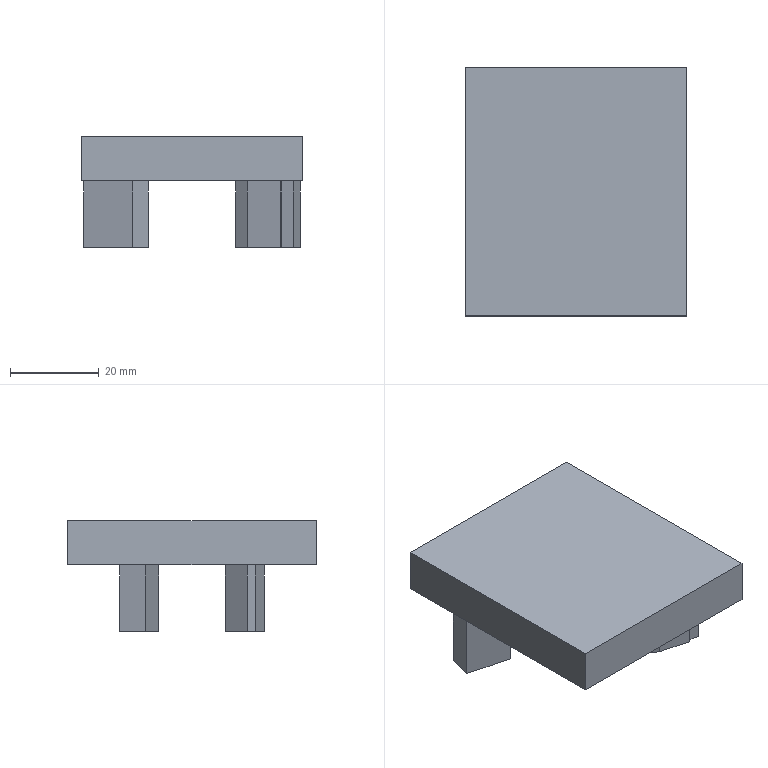Component | SolidWorks | 2023-12-12-30-1 | 1 solid | 22 faces | box 50 x 56 x 25 mm | volume 30440 mm3 | plane 22 | material S45C
build123d program:
from build123d import *

# Parameters (mm, degrees)
SKETCH1_W           = 50
SKETCH1_H           = 56
BOSS_EXTRUDE1_DEPTH = 25
SKETCH2_W           = 50
SKETCH2_H           = 56
CUT_EXTRUDE1_DEPTH  = 15


with BuildPart() as part:
    # Sketch1 → Boss-Extrude1 (new body)
    with BuildSketch(Plane.XY):
        with Locations((25, 28)):
            Rectangle(SKETCH1_W, SKETCH1_H)
    extrude(amount=BOSS_EXTRUDE1_DEPTH)

    # Sketch2 → Cut-Extrude1 (cut)
    with BuildSketch(Plane(origin=(0, 0, 0), x_dir=(-1, 0, 0), z_dir=(0, 0, -1))):
        with Locations((-25, 28)):
            Rectangle(SKETCH2_W, SKETCH2_H)
        Polygon((-44.917, 11.713), (-37.417, 13.723), (-34.917, 15.473), (-38.4, 20.447), (-49.4, 17.5), (-47.847, 11.704), (-45.111, 12.438), align=None, mode=Mode.SUBTRACT)
        Polygon((-4.889, 43.562), (-5.083, 44.287), (-12.583, 42.277), (-15.083, 40.527), (-11.6, 35.553), (-0.6, 38.5), (-2.153, 44.296), align=None, mode=Mode.SUBTRACT)
    extrude(amount=-CUT_EXTRUDE1_DEPTH, mode=Mode.SUBTRACT)


solid = part.part

# Placed as in the assembly
solid = solid.moved(Location((-93.778, -30.867, 92.891), (0, 0, 0)))
STEP:
#1=COLOUR_RGB('',0.7922,0.8196,0.9333);
#2=FILL_AREA_STYLE_COLOUR('',#1);
#3=FILL_AREA_STYLE('',(#2));
#4=SURFACE_STYLE_FILL_AREA(#3);
#5=SURFACE_SIDE_STYLE('',(#4));
#6=SURFACE_STYLE_USAGE(.BOTH.,#5);
#7=PRESENTATION_STYLE_ASSIGNMENT((#6));
#8=CARTESIAN_POINT('',(-3.692,0.9895,4.641));
#9=VERTEX_POINT('',#8);
#10=CARTESIAN_POINT('',(-3.692,0.9895,4.248));
#11=VERTEX_POINT('',#10);
#12=CARTESIAN_POINT('',(-3.692,0.9895,4.641));
#13=DIRECTION('',(0.,0.,-1.));
#14=VECTOR('',#13,39.37);
#15=LINE('',#12,#14);
#16=EDGE_CURVE('',#9,#11,#15,.T.);
#17=ORIENTED_EDGE('',*,*,#16,.T.);
#18=CARTESIAN_POINT('',(-3.692,-1.215,4.248));
#19=VERTEX_POINT('',#18);
#20=CARTESIAN_POINT('',(-3.692,-1.215,4.248));
#21=DIRECTION('',(0.,1.,0.));
#22=VECTOR('',#21,39.37);
#23=LINE('',#20,#22);
#24=EDGE_CURVE('',#19,#11,#23,.T.);
#25=ORIENTED_EDGE('',*,*,#24,.F.);
#26=CARTESIAN_POINT('',(-3.692,-1.215,4.641));
#27=VERTEX_POINT('',#26);
#28=CARTESIAN_POINT('',(-3.692,-1.215,4.641));
#29=DIRECTION('',(0.,0.,-1.));
#30=VECTOR('',#29,39.37);
#31=LINE('',#28,#30);
#32=EDGE_CURVE('',#27,#19,#31,.T.);
#33=ORIENTED_EDGE('',*,*,#32,.F.);
#34=CARTESIAN_POINT('',(-3.692,-1.215,4.641));
#35=DIRECTION('',(0.,-1.,0.));
#36=VECTOR('',#35,39.37);
#37=LINE('',#34,#36);
#38=EDGE_CURVE('',#9,#27,#37,.T.);
#39=ORIENTED_EDGE('',*,*,#38,.F.);
#40=EDGE_LOOP('',(#17,#25,#33,#39));
#41=FACE_OUTER_BOUND('',#40,.T.);
#42=CARTESIAN_POINT('',(-3.692,-1.215,4.641));
#43=DIRECTION('',(1.,0.,0.));
#44=DIRECTION('',(0.,0.,-1.));
#45=AXIS2_PLACEMENT_3D('',#42,#43,#44);
#46=PLANE('',#45);
#47=ADVANCED_FACE('',(#41),#46,.F.);
#48=ORIENTED_EDGE('',*,*,#32,.T.);
#49=CARTESIAN_POINT('',(-1.724,-1.215,4.248));
#50=VERTEX_POINT('',#49);
#51=CARTESIAN_POINT('',(-1.724,-1.215,4.248));
#52=DIRECTION('',(-1.,0.,0.));
#53=VECTOR('',#52,39.37);
#54=LINE('',#51,#53);
#55=EDGE_CURVE('',#50,#19,#54,.T.);
#56=ORIENTED_EDGE('',*,*,#55,.F.);
#57=CARTESIAN_POINT('',(-1.724,-1.215,4.641));
#58=VERTEX_POINT('',#57);
#59=CARTESIAN_POINT('',(-1.724,-1.215,4.641));
#60=DIRECTION('',(0.,0.,-1.));
#61=VECTOR('',#60,39.37);
#62=LINE('',#59,#61);
#63=EDGE_CURVE('',#58,#50,#62,.T.);
#64=ORIENTED_EDGE('',*,*,#63,.F.);
#65=CARTESIAN_POINT('',(-3.692,-1.215,4.641));
#66=DIRECTION('',(1.,0.,0.));
#67=VECTOR('',#66,39.37);
#68=LINE('',#65,#67);
#69=EDGE_CURVE('',#27,#58,#68,.T.);
#70=ORIENTED_EDGE('',*,*,#69,.F.);
#71=EDGE_LOOP('',(#48,#56,#64,#70));
#72=FACE_OUTER_BOUND('',#71,.T.);
#73=CARTESIAN_POINT('',(-3.692,-1.215,4.641));
#74=DIRECTION('',(0.,1.,0.));
#75=DIRECTION('',(0.,0.,1.));
#76=AXIS2_PLACEMENT_3D('',#73,#74,#75);
#77=PLANE('',#76);
#78=ADVANCED_FACE('',(#72),#77,.F.);
#79=ORIENTED_EDGE('',*,*,#63,.T.);
#80=CARTESIAN_POINT('',(-1.724,0.9895,4.248));
#81=VERTEX_POINT('',#80);
#82=CARTESIAN_POINT('',(-1.724,-1.215,4.248));
#83=DIRECTION('',(0.,-1.,0.));
#84=VECTOR('',#83,39.37);
#85=LINE('',#82,#84);
#86=EDGE_CURVE('',#81,#50,#85,.T.);
#87=ORIENTED_EDGE('',*,*,#86,.F.);
#88=CARTESIAN_POINT('',(-1.724,0.9895,4.641));
#89=VERTEX_POINT('',#88);
#90=CARTESIAN_POINT('',(-1.724,0.9895,4.641));
#91=DIRECTION('',(0.,0.,-1.));
#92=VECTOR('',#91,39.37);
#93=LINE('',#90,#92);
#94=EDGE_CURVE('',#89,#81,#93,.T.);
#95=ORIENTED_EDGE('',*,*,#94,.F.);
#96=CARTESIAN_POINT('',(-1.724,-1.215,4.641));
#97=DIRECTION('',(0.,1.,0.));
#98=VECTOR('',#97,39.37);
#99=LINE('',#96,#98);
#100=EDGE_CURVE('',#58,#89,#99,.T.);
#101=ORIENTED_EDGE('',*,*,#100,.F.);
#102=EDGE_LOOP('',(#79,#87,#95,#101));
#103=FACE_OUTER_BOUND('',#102,.T.);
#104=CARTESIAN_POINT('',(-1.724,-1.215,4.641));
#105=DIRECTION('',(-1.,0.,0.));
#106=DIRECTION('',(0.,0.,1.));
#107=AXIS2_PLACEMENT_3D('',#104,#105,#106);
#108=PLANE('',#107);
#109=ADVANCED_FACE('',(#103),#108,.F.);
#110=ORIENTED_EDGE('',*,*,#94,.T.);
#111=CARTESIAN_POINT('',(-1.724,0.9895,4.248));
#112=DIRECTION('',(1.,0.,0.));
#113=VECTOR('',#112,39.37);
#114=LINE('',#111,#113);
#115=EDGE_CURVE('',#11,#81,#114,.T.);
#116=ORIENTED_EDGE('',*,*,#115,.F.);
#117=ORIENTED_EDGE('',*,*,#16,.F.);
#118=CARTESIAN_POINT('',(-3.692,0.9895,4.641));
#119=DIRECTION('',(-1.,0.,0.));
#120=VECTOR('',#119,39.37);
#121=LINE('',#118,#120);
#122=EDGE_CURVE('',#89,#9,#121,.T.);
#123=ORIENTED_EDGE('',*,*,#122,.F.);
#124=EDGE_LOOP('',(#110,#116,#117,#123));
#125=FACE_OUTER_BOUND('',#124,.T.);
#126=CARTESIAN_POINT('',(-3.692,0.9895,4.641));
#127=DIRECTION('',(0.,-1.,0.));
#128=DIRECTION('',(0.,0.,-1.));
#129=AXIS2_PLACEMENT_3D('',#126,#127,#128);
#130=PLANE('',#129);
#131=ADVANCED_FACE('',(#125),#130,.F.);
#132=ORIENTED_EDGE('',*,*,#38,.T.);
#133=ORIENTED_EDGE('',*,*,#69,.T.);
#134=ORIENTED_EDGE('',*,*,#100,.T.);
#135=ORIENTED_EDGE('',*,*,#122,.T.);
#136=EDGE_LOOP('',(#132,#133,#134,#135));
#137=FACE_OUTER_BOUND('',#136,.T.);
#138=CARTESIAN_POINT('',(-3.692,-1.215,4.641));
#139=DIRECTION('',(0.,0.,-1.));
#140=DIRECTION('',(-1.,0.,0.));
#141=AXIS2_PLACEMENT_3D('',#138,#139,#140);
#142=PLANE('',#141);
#143=ADVANCED_FACE('',(#137),#142,.F.);
#144=CARTESIAN_POINT('',(-3.492,0.5284,4.248));
#145=VERTEX_POINT('',#144);
#146=CARTESIAN_POINT('',(-3.197,0.4492,4.248));
#147=VERTEX_POINT('',#146);
#148=CARTESIAN_POINT('',(-3.492,0.5284,4.248));
#149=DIRECTION('',(0.9659,-0.2588,0.));
#150=VECTOR('',#149,39.37);
#151=LINE('',#148,#150);
#152=EDGE_CURVE('',#145,#147,#151,.T.);
#153=ORIENTED_EDGE('',*,*,#152,.F.);
#154=CARTESIAN_POINT('',(-3.5,0.4998,4.248));
#155=VERTEX_POINT('',#154);
#156=CARTESIAN_POINT('',(-3.5,0.4998,4.248));
#157=DIRECTION('',(0.2588,0.9659,0.));
#158=VECTOR('',#157,39.37);
#159=LINE('',#156,#158);
#160=EDGE_CURVE('',#155,#145,#159,.T.);
#161=ORIENTED_EDGE('',*,*,#160,.F.);
#162=CARTESIAN_POINT('',(-3.607,0.5287,4.248));
#163=VERTEX_POINT('',#162);
#164=CARTESIAN_POINT('',(-3.607,0.5287,4.248));
#165=DIRECTION('',(0.9659,-0.2588,0.));
#166=VECTOR('',#165,39.37);
#167=LINE('',#164,#166);
#168=EDGE_CURVE('',#163,#155,#167,.T.);
#169=ORIENTED_EDGE('',*,*,#168,.F.);
#170=CARTESIAN_POINT('',(-3.668,0.3005,4.248));
#171=VERTEX_POINT('',#170);
#172=CARTESIAN_POINT('',(-3.668,0.3005,4.248));
#173=DIRECTION('',(0.2588,0.9659,0.));
#174=VECTOR('',#173,39.37);
#175=LINE('',#172,#174);
#176=EDGE_CURVE('',#171,#163,#175,.T.);
#177=ORIENTED_EDGE('',*,*,#176,.F.);
#178=CARTESIAN_POINT('',(-3.235,0.1845,4.248));
#179=VERTEX_POINT('',#178);
#180=CARTESIAN_POINT('',(-3.235,0.1845,4.248));
#181=DIRECTION('',(-0.9659,0.2588,0.));
#182=VECTOR('',#181,39.37);
#183=LINE('',#180,#182);
#184=EDGE_CURVE('',#179,#171,#183,.T.);
#185=ORIENTED_EDGE('',*,*,#184,.F.);
#186=CARTESIAN_POINT('',(-3.098,0.3803,4.248));
#187=VERTEX_POINT('',#186);
#188=CARTESIAN_POINT('',(-3.098,0.3803,4.248));
#189=DIRECTION('',(-0.5736,-0.8192,0.));
#190=VECTOR('',#189,39.37);
#191=LINE('',#188,#190);
#192=EDGE_CURVE('',#187,#179,#191,.T.);
#193=ORIENTED_EDGE('',*,*,#192,.F.);
#194=CARTESIAN_POINT('',(-3.197,0.4492,4.248));
#195=DIRECTION('',(0.8192,-0.5736,0.));
#196=VECTOR('',#195,39.37);
#197=LINE('',#194,#196);
#198=EDGE_CURVE('',#147,#187,#197,.T.);
#199=ORIENTED_EDGE('',*,*,#198,.F.);
#200=EDGE_LOOP('',(#153,#161,#169,#177,#185,#193,#199));
#201=FACE_BOUND('',#200,.T.);
#202=CARTESIAN_POINT('',(-1.916,-0.7256,4.248));
#203=VERTEX_POINT('',#202);
#204=CARTESIAN_POINT('',(-1.924,-0.7541,4.248));
#205=VERTEX_POINT('',#204);
#206=CARTESIAN_POINT('',(-1.916,-0.7256,4.248));
#207=DIRECTION('',(-0.2588,-0.9659,0.));
#208=VECTOR('',#207,39.37);
#209=LINE('',#206,#208);
#210=EDGE_CURVE('',#203,#205,#209,.T.);
#211=ORIENTED_EDGE('',*,*,#210,.F.);
#212=CARTESIAN_POINT('',(-1.808,-0.7544,4.248));
#213=VERTEX_POINT('',#212);
#214=CARTESIAN_POINT('',(-1.808,-0.7544,4.248));
#215=DIRECTION('',(-0.9659,0.2588,0.));
#216=VECTOR('',#215,39.37);
#217=LINE('',#214,#216);
#218=EDGE_CURVE('',#213,#203,#217,.T.);
#219=ORIENTED_EDGE('',*,*,#218,.F.);
#220=CARTESIAN_POINT('',(-1.747,-0.5262,4.248));
#221=VERTEX_POINT('',#220);
#222=CARTESIAN_POINT('',(-1.747,-0.5262,4.248));
#223=DIRECTION('',(-0.2588,-0.9659,0.));
#224=VECTOR('',#223,39.37);
#225=LINE('',#222,#224);
#226=EDGE_CURVE('',#221,#213,#225,.T.);
#227=ORIENTED_EDGE('',*,*,#226,.F.);
#228=CARTESIAN_POINT('',(-2.18,-0.4102,4.248));
#229=VERTEX_POINT('',#228);
#230=CARTESIAN_POINT('',(-2.18,-0.4102,4.248));
#231=DIRECTION('',(0.9659,-0.2588,0.));
#232=VECTOR('',#231,39.37);
#233=LINE('',#230,#232);
#234=EDGE_CURVE('',#229,#221,#233,.T.);
#235=ORIENTED_EDGE('',*,*,#234,.F.);
#236=CARTESIAN_POINT('',(-2.317,-0.606,4.248));
#237=VERTEX_POINT('',#236);
#238=CARTESIAN_POINT('',(-2.317,-0.606,4.248));
#239=DIRECTION('',(0.5736,0.8192,0.));
#240=VECTOR('',#239,39.37);
#241=LINE('',#238,#240);
#242=EDGE_CURVE('',#237,#229,#241,.T.);
#243=ORIENTED_EDGE('',*,*,#242,.F.);
#244=CARTESIAN_POINT('',(-2.219,-0.675,4.248));
#245=VERTEX_POINT('',#244);
#246=CARTESIAN_POINT('',(-2.219,-0.675,4.248));
#247=DIRECTION('',(-0.8192,0.5736,0.));
#248=VECTOR('',#247,39.37);
#249=LINE('',#246,#248);
#250=EDGE_CURVE('',#245,#237,#249,.T.);
#251=ORIENTED_EDGE('',*,*,#250,.F.);
#252=CARTESIAN_POINT('',(-1.924,-0.7541,4.248));
#253=DIRECTION('',(-0.9659,0.2588,0.));
#254=VECTOR('',#253,39.37);
#255=LINE('',#252,#254);
#256=EDGE_CURVE('',#205,#245,#255,.T.);
#257=ORIENTED_EDGE('',*,*,#256,.F.);
#258=EDGE_LOOP('',(#211,#219,#227,#235,#243,#251,#257));
#259=FACE_BOUND('',#258,.T.);
#260=ORIENTED_EDGE('',*,*,#86,.T.);
#261=ORIENTED_EDGE('',*,*,#55,.T.);
#262=ORIENTED_EDGE('',*,*,#24,.T.);
#263=ORIENTED_EDGE('',*,*,#115,.T.);
#264=EDGE_LOOP('',(#260,#261,#262,#263));
#265=FACE_OUTER_BOUND('',#264,.T.);
#266=CARTESIAN_POINT('',(-3.692,-1.215,4.248));
#267=DIRECTION('',(0.,0.,1.));
#268=DIRECTION('',(1.,0.,0.));
#269=AXIS2_PLACEMENT_3D('',#266,#267,#268);
#270=PLANE('',#269);
#271=ADVANCED_FACE('',(#201,#259,#265),#270,.F.);
#272=CARTESIAN_POINT('',(-1.916,-0.7256,3.657));
#273=VERTEX_POINT('',#272);
#274=CARTESIAN_POINT('',(-1.924,-0.7541,3.657));
#275=VERTEX_POINT('',#274);
#276=CARTESIAN_POINT('',(-1.916,-0.7256,3.657));
#277=DIRECTION('',(-0.2588,-0.9659,0.));
#278=VECTOR('',#277,39.37);
#279=LINE('',#276,#278);
#280=EDGE_CURVE('',#273,#275,#279,.T.);
#281=ORIENTED_EDGE('',*,*,#280,.F.);
#282=CARTESIAN_POINT('',(-1.916,-0.7256,4.248));
#283=DIRECTION('',(0.,0.,-1.));
#284=VECTOR('',#283,39.37);
#285=LINE('',#282,#284);
#286=EDGE_CURVE('',#203,#273,#285,.T.);
#287=ORIENTED_EDGE('',*,*,#286,.F.);
#288=ORIENTED_EDGE('',*,*,#210,.T.);
#289=CARTESIAN_POINT('',(-1.924,-0.7541,4.248));
#290=DIRECTION('',(0.,0.,-1.));
#291=VECTOR('',#290,39.37);
#292=LINE('',#289,#291);
#293=EDGE_CURVE('',#205,#275,#292,.T.);
#294=ORIENTED_EDGE('',*,*,#293,.T.);
#295=EDGE_LOOP('',(#281,#287,#288,#294));
#296=FACE_OUTER_BOUND('',#295,.T.);
#297=CARTESIAN_POINT('',(-1.916,-0.7256,4.248));
#298=DIRECTION('',(0.9659,-0.2588,0.));
#299=DIRECTION('',(0.2588,0.9659,0.));
#300=AXIS2_PLACEMENT_3D('',#297,#298,#299);
#301=PLANE('',#300);
#302=ADVANCED_FACE('',(#296),#301,.T.);
#303=CARTESIAN_POINT('',(-1.808,-0.7544,3.657));
#304=VERTEX_POINT('',#303);
#305=CARTESIAN_POINT('',(-1.808,-0.7544,3.657));
#306=DIRECTION('',(-0.9659,0.2588,0.));
#307=VECTOR('',#306,39.37);
#308=LINE('',#305,#307);
#309=EDGE_CURVE('',#304,#273,#308,.T.);
#310=ORIENTED_EDGE('',*,*,#309,.F.);
#311=CARTESIAN_POINT('',(-1.808,-0.7544,4.248));
#312=DIRECTION('',(0.,0.,-1.));
#313=VECTOR('',#312,39.37);
#314=LINE('',#311,#313);
#315=EDGE_CURVE('',#213,#304,#314,.T.);
#316=ORIENTED_EDGE('',*,*,#315,.F.);
#317=ORIENTED_EDGE('',*,*,#218,.T.);
#318=ORIENTED_EDGE('',*,*,#286,.T.);
#319=EDGE_LOOP('',(#310,#316,#317,#318));
#320=FACE_OUTER_BOUND('',#319,.T.);
#321=CARTESIAN_POINT('',(-1.808,-0.7544,4.248));
#322=DIRECTION('',(-0.2588,-0.9659,0.));
#323=DIRECTION('',(0.9659,-0.2588,0.));
#324=AXIS2_PLACEMENT_3D('',#321,#322,#323);
#325=PLANE('',#324);
#326=ADVANCED_FACE('',(#320),#325,.T.);
#327=CARTESIAN_POINT('',(-1.747,-0.5262,3.657));
#328=VERTEX_POINT('',#327);
#329=CARTESIAN_POINT('',(-1.747,-0.5262,3.657));
#330=DIRECTION('',(-0.2588,-0.9659,0.));
#331=VECTOR('',#330,39.37);
#332=LINE('',#329,#331);
#333=EDGE_CURVE('',#328,#304,#332,.T.);
#334=ORIENTED_EDGE('',*,*,#333,.F.);
#335=CARTESIAN_POINT('',(-1.747,-0.5262,4.248));
#336=DIRECTION('',(0.,0.,-1.));
#337=VECTOR('',#336,39.37);
#338=LINE('',#335,#337);
#339=EDGE_CURVE('',#221,#328,#338,.T.);
#340=ORIENTED_EDGE('',*,*,#339,.F.);
#341=ORIENTED_EDGE('',*,*,#226,.T.);
#342=ORIENTED_EDGE('',*,*,#315,.T.);
#343=EDGE_LOOP('',(#334,#340,#341,#342));
#344=FACE_OUTER_BOUND('',#343,.T.);
#345=CARTESIAN_POINT('',(-1.747,-0.5262,4.248));
#346=DIRECTION('',(0.9659,-0.2588,0.));
#347=DIRECTION('',(0.2588,0.9659,0.));
#348=AXIS2_PLACEMENT_3D('',#345,#346,#347);
#349=PLANE('',#348);
#350=ADVANCED_FACE('',(#344),#349,.T.);
#351=CARTESIAN_POINT('',(-2.18,-0.4102,3.657));
#352=VERTEX_POINT('',#351);
#353=CARTESIAN_POINT('',(-2.18,-0.4102,3.657));
#354=DIRECTION('',(0.9659,-0.2588,0.));
#355=VECTOR('',#354,39.37);
#356=LINE('',#353,#355);
#357=EDGE_CURVE('',#352,#328,#356,.T.);
#358=ORIENTED_EDGE('',*,*,#357,.F.);
#359=CARTESIAN_POINT('',(-2.18,-0.4102,4.248));
#360=DIRECTION('',(0.,0.,-1.));
#361=VECTOR('',#360,39.37);
#362=LINE('',#359,#361);
#363=EDGE_CURVE('',#229,#352,#362,.T.);
#364=ORIENTED_EDGE('',*,*,#363,.F.);
#365=ORIENTED_EDGE('',*,*,#234,.T.);
#366=ORIENTED_EDGE('',*,*,#339,.T.);
#367=EDGE_LOOP('',(#358,#364,#365,#366));
#368=FACE_OUTER_BOUND('',#367,.T.);
#369=CARTESIAN_POINT('',(-2.18,-0.4102,4.248));
#370=DIRECTION('',(0.2588,0.9659,0.));
#371=DIRECTION('',(-0.9659,0.2588,0.));
#372=AXIS2_PLACEMENT_3D('',#369,#370,#371);
#373=PLANE('',#372);
#374=ADVANCED_FACE('',(#368),#373,.T.);
#375=CARTESIAN_POINT('',(-2.317,-0.606,3.657));
#376=VERTEX_POINT('',#375);
#377=CARTESIAN_POINT('',(-2.317,-0.606,3.657));
#378=DIRECTION('',(0.5736,0.8192,0.));
#379=VECTOR('',#378,39.37);
#380=LINE('',#377,#379);
#381=EDGE_CURVE('',#376,#352,#380,.T.);
#382=ORIENTED_EDGE('',*,*,#381,.F.);
#383=CARTESIAN_POINT('',(-2.317,-0.606,4.248));
#384=DIRECTION('',(0.,0.,-1.));
#385=VECTOR('',#384,39.37);
#386=LINE('',#383,#385);
#387=EDGE_CURVE('',#237,#376,#386,.T.);
#388=ORIENTED_EDGE('',*,*,#387,.F.);
#389=ORIENTED_EDGE('',*,*,#242,.T.);
#390=ORIENTED_EDGE('',*,*,#363,.T.);
#391=EDGE_LOOP('',(#382,#388,#389,#390));
#392=FACE_OUTER_BOUND('',#391,.T.);
#393=CARTESIAN_POINT('',(-2.317,-0.606,4.248));
#394=DIRECTION('',(-0.8192,0.5736,0.));
#395=DIRECTION('',(-0.5736,-0.8192,0.));
#396=AXIS2_PLACEMENT_3D('',#393,#394,#395);
#397=PLANE('',#396);
#398=ADVANCED_FACE('',(#392),#397,.T.);
#399=CARTESIAN_POINT('',(-2.219,-0.675,3.657));
#400=VERTEX_POINT('',#399);
#401=CARTESIAN_POINT('',(-2.219,-0.675,3.657));
#402=DIRECTION('',(-0.8192,0.5736,0.));
#403=VECTOR('',#402,39.37);
#404=LINE('',#401,#403);
#405=EDGE_CURVE('',#400,#376,#404,.T.);
#406=ORIENTED_EDGE('',*,*,#405,.F.);
#407=CARTESIAN_POINT('',(-2.219,-0.675,4.248));
#408=DIRECTION('',(0.,0.,-1.));
#409=VECTOR('',#408,39.37);
#410=LINE('',#407,#409);
#411=EDGE_CURVE('',#245,#400,#410,.T.);
#412=ORIENTED_EDGE('',*,*,#411,.F.);
#413=ORIENTED_EDGE('',*,*,#250,.T.);
#414=ORIENTED_EDGE('',*,*,#387,.T.);
#415=EDGE_LOOP('',(#406,#412,#413,#414));
#416=FACE_OUTER_BOUND('',#415,.T.);
#417=CARTESIAN_POINT('',(-2.219,-0.675,4.248));
#418=DIRECTION('',(-0.5736,-0.8192,0.));
#419=DIRECTION('',(0.8192,-0.5736,0.));
#420=AXIS2_PLACEMENT_3D('',#417,#418,#419);
#421=PLANE('',#420);
#422=ADVANCED_FACE('',(#416),#421,.T.);
#423=CARTESIAN_POINT('',(-1.924,-0.7541,3.657));
#424=DIRECTION('',(-0.9659,0.2588,0.));
#425=VECTOR('',#424,39.37);
#426=LINE('',#423,#425);
#427=EDGE_CURVE('',#275,#400,#426,.T.);
#428=ORIENTED_EDGE('',*,*,#427,.F.);
#429=ORIENTED_EDGE('',*,*,#293,.F.);
#430=ORIENTED_EDGE('',*,*,#256,.T.);
#431=ORIENTED_EDGE('',*,*,#411,.T.);
#432=EDGE_LOOP('',(#428,#429,#430,#431));
#433=FACE_OUTER_BOUND('',#432,.T.);
#434=CARTESIAN_POINT('',(-1.924,-0.7541,4.248));
#435=DIRECTION('',(-0.2588,-0.9659,0.));
#436=DIRECTION('',(0.9659,-0.2588,0.));
#437=AXIS2_PLACEMENT_3D('',#434,#435,#436);
#438=PLANE('',#437);
#439=ADVANCED_FACE('',(#433),#438,.T.);
#440=CARTESIAN_POINT('',(-3.492,0.5284,3.657));
#441=VERTEX_POINT('',#440);
#442=CARTESIAN_POINT('',(-3.197,0.4492,3.657));
#443=VERTEX_POINT('',#442);
#444=CARTESIAN_POINT('',(-3.492,0.5284,3.657));
#445=DIRECTION('',(0.9659,-0.2588,0.));
#446=VECTOR('',#445,39.37);
#447=LINE('',#444,#446);
#448=EDGE_CURVE('',#441,#443,#447,.T.);
#449=ORIENTED_EDGE('',*,*,#448,.F.);
#450=CARTESIAN_POINT('',(-3.492,0.5284,4.248));
#451=DIRECTION('',(0.,0.,-1.));
#452=VECTOR('',#451,39.37);
#453=LINE('',#450,#452);
#454=EDGE_CURVE('',#145,#441,#453,.T.);
#455=ORIENTED_EDGE('',*,*,#454,.F.);
#456=ORIENTED_EDGE('',*,*,#152,.T.);
#457=CARTESIAN_POINT('',(-3.197,0.4492,4.248));
#458=DIRECTION('',(0.,0.,-1.));
#459=VECTOR('',#458,39.37);
#460=LINE('',#457,#459);
#461=EDGE_CURVE('',#147,#443,#460,.T.);
#462=ORIENTED_EDGE('',*,*,#461,.T.);
#463=EDGE_LOOP('',(#449,#455,#456,#462));
#464=FACE_OUTER_BOUND('',#463,.T.);
#465=CARTESIAN_POINT('',(-3.492,0.5284,4.248));
#466=DIRECTION('',(0.2588,0.9659,0.));
#467=DIRECTION('',(-0.9659,0.2588,0.));
#468=AXIS2_PLACEMENT_3D('',#465,#466,#467);
#469=PLANE('',#468);
#470=ADVANCED_FACE('',(#464),#469,.T.);
#471=CARTESIAN_POINT('',(-3.5,0.4998,3.657));
#472=VERTEX_POINT('',#471);
#473=CARTESIAN_POINT('',(-3.5,0.4998,3.657));
#474=DIRECTION('',(0.2588,0.9659,0.));
#475=VECTOR('',#474,39.37);
#476=LINE('',#473,#475);
#477=EDGE_CURVE('',#472,#441,#476,.T.);
#478=ORIENTED_EDGE('',*,*,#477,.F.);
#479=CARTESIAN_POINT('',(-3.5,0.4998,4.248));
#480=DIRECTION('',(0.,0.,-1.));
#481=VECTOR('',#480,39.37);
#482=LINE('',#479,#481);
#483=EDGE_CURVE('',#155,#472,#482,.T.);
#484=ORIENTED_EDGE('',*,*,#483,.F.);
#485=ORIENTED_EDGE('',*,*,#160,.T.);
#486=ORIENTED_EDGE('',*,*,#454,.T.);
#487=EDGE_LOOP('',(#478,#484,#485,#486));
#488=FACE_OUTER_BOUND('',#487,.T.);
#489=CARTESIAN_POINT('',(-3.5,0.4998,4.248));
#490=DIRECTION('',(-0.9659,0.2588,0.));
#491=DIRECTION('',(-0.2588,-0.9659,0.));
#492=AXIS2_PLACEMENT_3D('',#489,#490,#491);
#493=PLANE('',#492);
#494=ADVANCED_FACE('',(#488),#493,.T.);
#495=CARTESIAN_POINT('',(-3.607,0.5287,3.657));
#496=VERTEX_POINT('',#495);
#497=CARTESIAN_POINT('',(-3.607,0.5287,3.657));
#498=DIRECTION('',(0.9659,-0.2588,0.));
#499=VECTOR('',#498,39.37);
#500=LINE('',#497,#499);
#501=EDGE_CURVE('',#496,#472,#500,.T.);
#502=ORIENTED_EDGE('',*,*,#501,.F.);
#503=CARTESIAN_POINT('',(-3.607,0.5287,4.248));
#504=DIRECTION('',(0.,0.,-1.));
#505=VECTOR('',#504,39.37);
#506=LINE('',#503,#505);
#507=EDGE_CURVE('',#163,#496,#506,.T.);
#508=ORIENTED_EDGE('',*,*,#507,.F.);
#509=ORIENTED_EDGE('',*,*,#168,.T.);
#510=ORIENTED_EDGE('',*,*,#483,.T.);
#511=EDGE_LOOP('',(#502,#508,#509,#510));
#512=FACE_OUTER_BOUND('',#511,.T.);
#513=CARTESIAN_POINT('',(-3.607,0.5287,4.248));
#514=DIRECTION('',(0.2588,0.9659,0.));
#515=DIRECTION('',(-0.9659,0.2588,0.));
#516=AXIS2_PLACEMENT_3D('',#513,#514,#515);
#517=PLANE('',#516);
#518=ADVANCED_FACE('',(#512),#517,.T.);
#519=CARTESIAN_POINT('',(-3.668,0.3005,3.657));
#520=VERTEX_POINT('',#519);
#521=CARTESIAN_POINT('',(-3.668,0.3005,3.657));
#522=DIRECTION('',(0.2588,0.9659,0.));
#523=VECTOR('',#522,39.37);
#524=LINE('',#521,#523);
#525=EDGE_CURVE('',#520,#496,#524,.T.);
#526=ORIENTED_EDGE('',*,*,#525,.F.);
#527=CARTESIAN_POINT('',(-3.668,0.3005,4.248));
#528=DIRECTION('',(0.,0.,-1.));
#529=VECTOR('',#528,39.37);
#530=LINE('',#527,#529);
#531=EDGE_CURVE('',#171,#520,#530,.T.);
#532=ORIENTED_EDGE('',*,*,#531,.F.);
#533=ORIENTED_EDGE('',*,*,#176,.T.);
#534=ORIENTED_EDGE('',*,*,#507,.T.);
#535=EDGE_LOOP('',(#526,#532,#533,#534));
#536=FACE_OUTER_BOUND('',#535,.T.);
#537=CARTESIAN_POINT('',(-3.668,0.3005,4.248));
#538=DIRECTION('',(-0.9659,0.2588,0.));
#539=DIRECTION('',(-0.2588,-0.9659,0.));
#540=AXIS2_PLACEMENT_3D('',#537,#538,#539);
#541=PLANE('',#540);
#542=ADVANCED_FACE('',(#536),#541,.T.);
#543=CARTESIAN_POINT('',(-3.235,0.1845,3.657));
#544=VERTEX_POINT('',#543);
#545=CARTESIAN_POINT('',(-3.235,0.1845,3.657));
#546=DIRECTION('',(-0.9659,0.2588,0.));
#547=VECTOR('',#546,39.37);
#548=LINE('',#545,#547);
#549=EDGE_CURVE('',#544,#520,#548,.T.);
#550=ORIENTED_EDGE('',*,*,#549,.F.);
#551=CARTESIAN_POINT('',(-3.235,0.1845,4.248));
#552=DIRECTION('',(0.,0.,-1.));
#553=VECTOR('',#552,39.37);
#554=LINE('',#551,#553);
#555=EDGE_CURVE('',#179,#544,#554,.T.);
#556=ORIENTED_EDGE('',*,*,#555,.F.);
#557=ORIENTED_EDGE('',*,*,#184,.T.);
#558=ORIENTED_EDGE('',*,*,#531,.T.);
#559=EDGE_LOOP('',(#550,#556,#557,#558));
#560=FACE_OUTER_BOUND('',#559,.T.);
#561=CARTESIAN_POINT('',(-3.235,0.1845,4.248));
#562=DIRECTION('',(-0.2588,-0.9659,0.));
#563=DIRECTION('',(0.9659,-0.2588,0.));
#564=AXIS2_PLACEMENT_3D('',#561,#562,#563);
#565=PLANE('',#564);
#566=ADVANCED_FACE('',(#560),#565,.T.);
#567=CARTESIAN_POINT('',(-3.098,0.3803,3.657));
#568=VERTEX_POINT('',#567);
#569=CARTESIAN_POINT('',(-3.098,0.3803,3.657));
#570=DIRECTION('',(-0.5736,-0.8192,0.));
#571=VECTOR('',#570,39.37);
#572=LINE('',#569,#571);
#573=EDGE_CURVE('',#568,#544,#572,.T.);
#574=ORIENTED_EDGE('',*,*,#573,.F.);
#575=CARTESIAN_POINT('',(-3.098,0.3803,4.248));
#576=DIRECTION('',(0.,0.,-1.));
#577=VECTOR('',#576,39.37);
#578=LINE('',#575,#577);
#579=EDGE_CURVE('',#187,#568,#578,.T.);
#580=ORIENTED_EDGE('',*,*,#579,.F.);
#581=ORIENTED_EDGE('',*,*,#192,.T.);
#582=ORIENTED_EDGE('',*,*,#555,.T.);
#583=EDGE_LOOP('',(#574,#580,#581,#582));
#584=FACE_OUTER_BOUND('',#583,.T.);
#585=CARTESIAN_POINT('',(-3.098,0.3803,4.248));
#586=DIRECTION('',(0.8192,-0.5736,0.));
#587=DIRECTION('',(0.5736,0.8192,0.));
#588=AXIS2_PLACEMENT_3D('',#585,#586,#587);
#589=PLANE('',#588);
#590=ADVANCED_FACE('',(#584),#589,.T.);
#591=CARTESIAN_POINT('',(-3.197,0.4492,3.657));
#592=DIRECTION('',(0.8192,-0.5736,0.));
#593=VECTOR('',#592,39.37);
#594=LINE('',#591,#593);
#595=EDGE_CURVE('',#443,#568,#594,.T.);
#596=ORIENTED_EDGE('',*,*,#595,.F.);
#597=ORIENTED_EDGE('',*,*,#461,.F.);
#598=ORIENTED_EDGE('',*,*,#198,.T.);
#599=ORIENTED_EDGE('',*,*,#579,.T.);
#600=EDGE_LOOP('',(#596,#597,#598,#599));
#601=FACE_OUTER_BOUND('',#600,.T.);
#602=CARTESIAN_POINT('',(-3.197,0.4492,4.248));
#603=DIRECTION('',(0.5736,0.8192,0.));
#604=DIRECTION('',(-0.8192,0.5736,0.));
#605=AXIS2_PLACEMENT_3D('',#602,#603,#604);
#606=PLANE('',#605);
#607=ADVANCED_FACE('',(#601),#606,.T.);
#608=ORIENTED_EDGE('',*,*,#309,.T.);
#609=ORIENTED_EDGE('',*,*,#280,.T.);
#610=ORIENTED_EDGE('',*,*,#427,.T.);
#611=ORIENTED_EDGE('',*,*,#405,.T.);
#612=ORIENTED_EDGE('',*,*,#381,.T.);
#613=ORIENTED_EDGE('',*,*,#357,.T.);
#614=ORIENTED_EDGE('',*,*,#333,.T.);
#615=EDGE_LOOP('',(#608,#609,#610,#611,#612,#613,#614));
#616=FACE_OUTER_BOUND('',#615,.T.);
#617=CARTESIAN_POINT('',(-3.692,-1.215,3.657));
#618=DIRECTION('',(0.,0.,-1.));
#619=DIRECTION('',(-1.,0.,0.));
#620=AXIS2_PLACEMENT_3D('',#617,#618,#619);
#621=PLANE('',#620);
#622=ADVANCED_FACE('',(#616),#621,.T.);
#623=ORIENTED_EDGE('',*,*,#477,.T.);
#624=ORIENTED_EDGE('',*,*,#448,.T.);
#625=ORIENTED_EDGE('',*,*,#595,.T.);
#626=ORIENTED_EDGE('',*,*,#573,.T.);
#627=ORIENTED_EDGE('',*,*,#549,.T.);
#628=ORIENTED_EDGE('',*,*,#525,.T.);
#629=ORIENTED_EDGE('',*,*,#501,.T.);
#630=EDGE_LOOP('',(#623,#624,#625,#626,#627,#628,#629));
#631=FACE_OUTER_BOUND('',#630,.T.);
#632=CARTESIAN_POINT('',(-3.692,-1.215,3.657));
#633=DIRECTION('',(0.,0.,-1.));
#634=DIRECTION('',(-1.,0.,0.));
#635=AXIS2_PLACEMENT_3D('',#632,#633,#634);
#636=PLANE('',#635);
#637=ADVANCED_FACE('',(#631),#636,.T.);
#638=CLOSED_SHELL('',(#47,#78,#109,#131,#143,#271,#302,#326,#350,#374,#398,#422,#439,#470,#494,#518,#542,#566,#590,#607,#622,#637));
#639=MANIFOLD_SOLID_BREP('',#638);
#640=STYLED_ITEM('',(#7),#639);
#641=PRESENTATION_LAYER_ASSIGNMENT('','',(#640));
#642=CARTESIAN_POINT('',(0.,0.,0.));
#643=DIRECTION('',(0.,0.,1.));
#644=DIRECTION('',(1.,0.,0.));
#645=AXIS2_PLACEMENT_3D('',#642,#643,#644);
#646=(LENGTH_UNIT()NAMED_UNIT(*)SI_UNIT($,.METRE.));
#647=LENGTH_MEASURE_WITH_UNIT(LENGTH_MEASURE(0.0254),#646);
#648=DIMENSIONAL_EXPONENTS(1.,0.,0.,0.,0.,0.,0.);
#649=(CONVERSION_BASED_UNIT('',#647)LENGTH_UNIT()NAMED_UNIT(#648));
#650=UNCERTAINTY_MEASURE_WITH_UNIT(LENGTH_MEASURE(0.00001),#649,'','');
#651=(NAMED_UNIT(*)PLANE_ANGLE_UNIT()SI_UNIT($,.RADIAN.));
#652=(NAMED_UNIT(*)SI_UNIT($,.STERADIAN.)SOLID_ANGLE_UNIT());
#653=(GEOMETRIC_REPRESENTATION_CONTEXT(3)GLOBAL_UNCERTAINTY_ASSIGNED_CONTEXT((#650))GLOBAL_UNIT_ASSIGNED_CONTEXT((#649,#651,#652))REPRESENTATION_CONTEXT('',''));
#654=ADVANCED_BREP_SHAPE_REPRESENTATION('',(#639,#645),#653);
#655=(LENGTH_UNIT()NAMED_UNIT(*)SI_UNIT($,.METRE.));
#656=LENGTH_MEASURE_WITH_UNIT(LENGTH_MEASURE(0.0254),#655);
#657=DIMENSIONAL_EXPONENTS(1.,0.,0.,0.,0.,0.,0.);
#658=(CONVERSION_BASED_UNIT('',#656)LENGTH_UNIT()NAMED_UNIT(#657));
#659=UNCERTAINTY_MEASURE_WITH_UNIT(LENGTH_MEASURE(0.00001),#658,'','');
#660=(NAMED_UNIT(*)PLANE_ANGLE_UNIT()SI_UNIT($,.RADIAN.));
#661=(NAMED_UNIT(*)SI_UNIT($,.STERADIAN.)SOLID_ANGLE_UNIT());
#662=(GEOMETRIC_REPRESENTATION_CONTEXT(3)GLOBAL_UNCERTAINTY_ASSIGNED_CONTEXT((#659))GLOBAL_UNIT_ASSIGNED_CONTEXT((#658,#660,#661))REPRESENTATION_CONTEXT('',''));
#663=MECHANICAL_DESIGN_GEOMETRIC_PRESENTATION_REPRESENTATION('',(#640),#662);